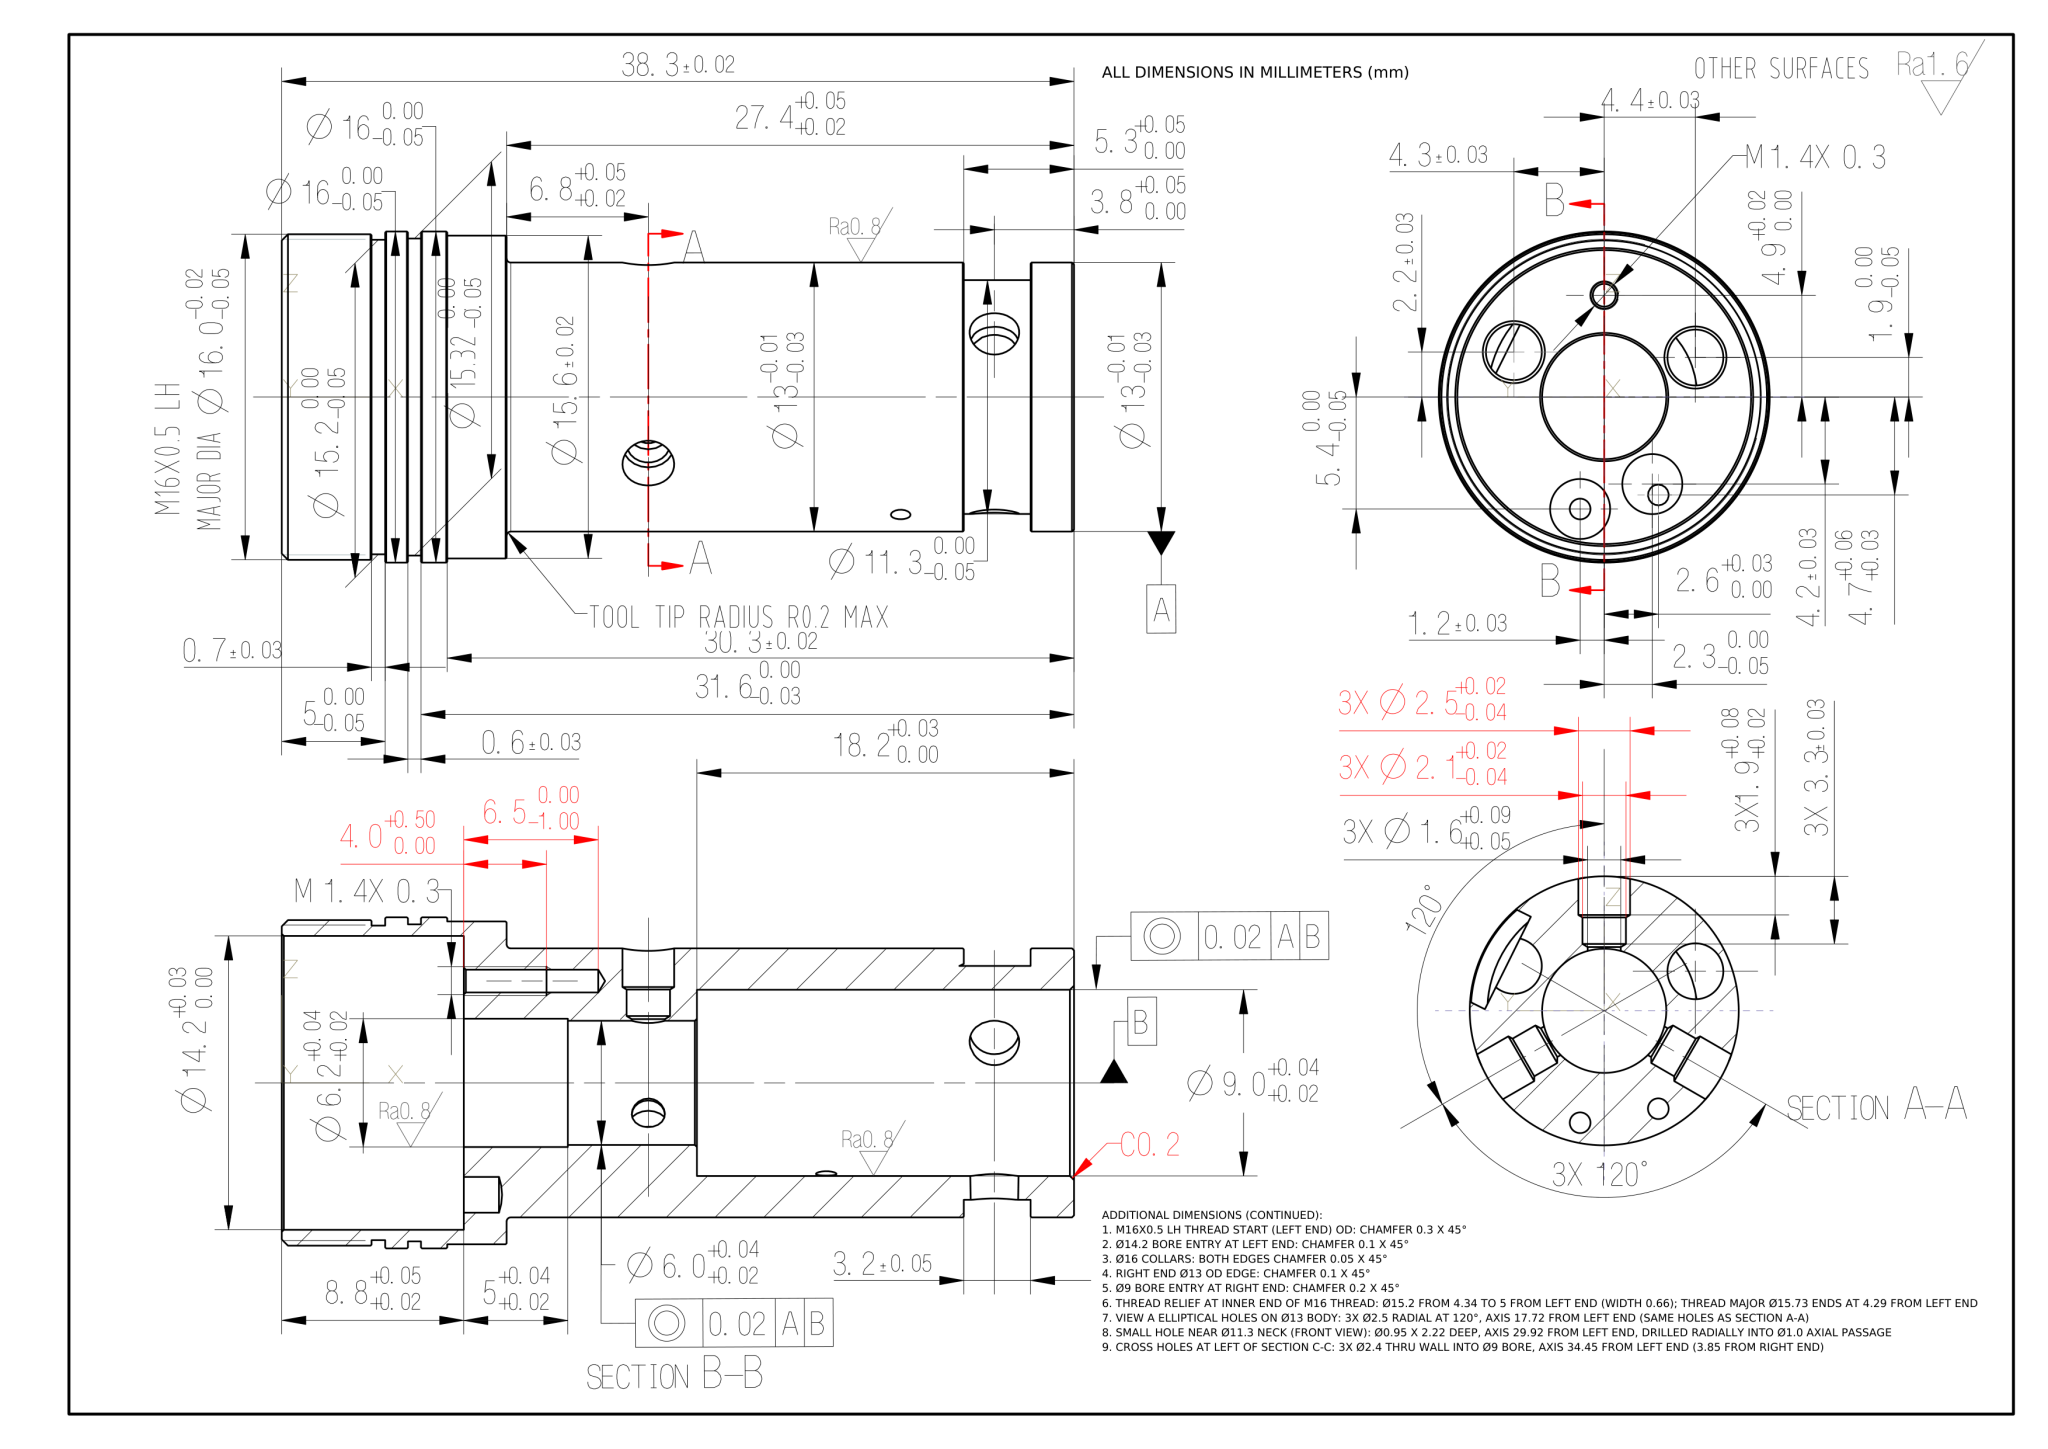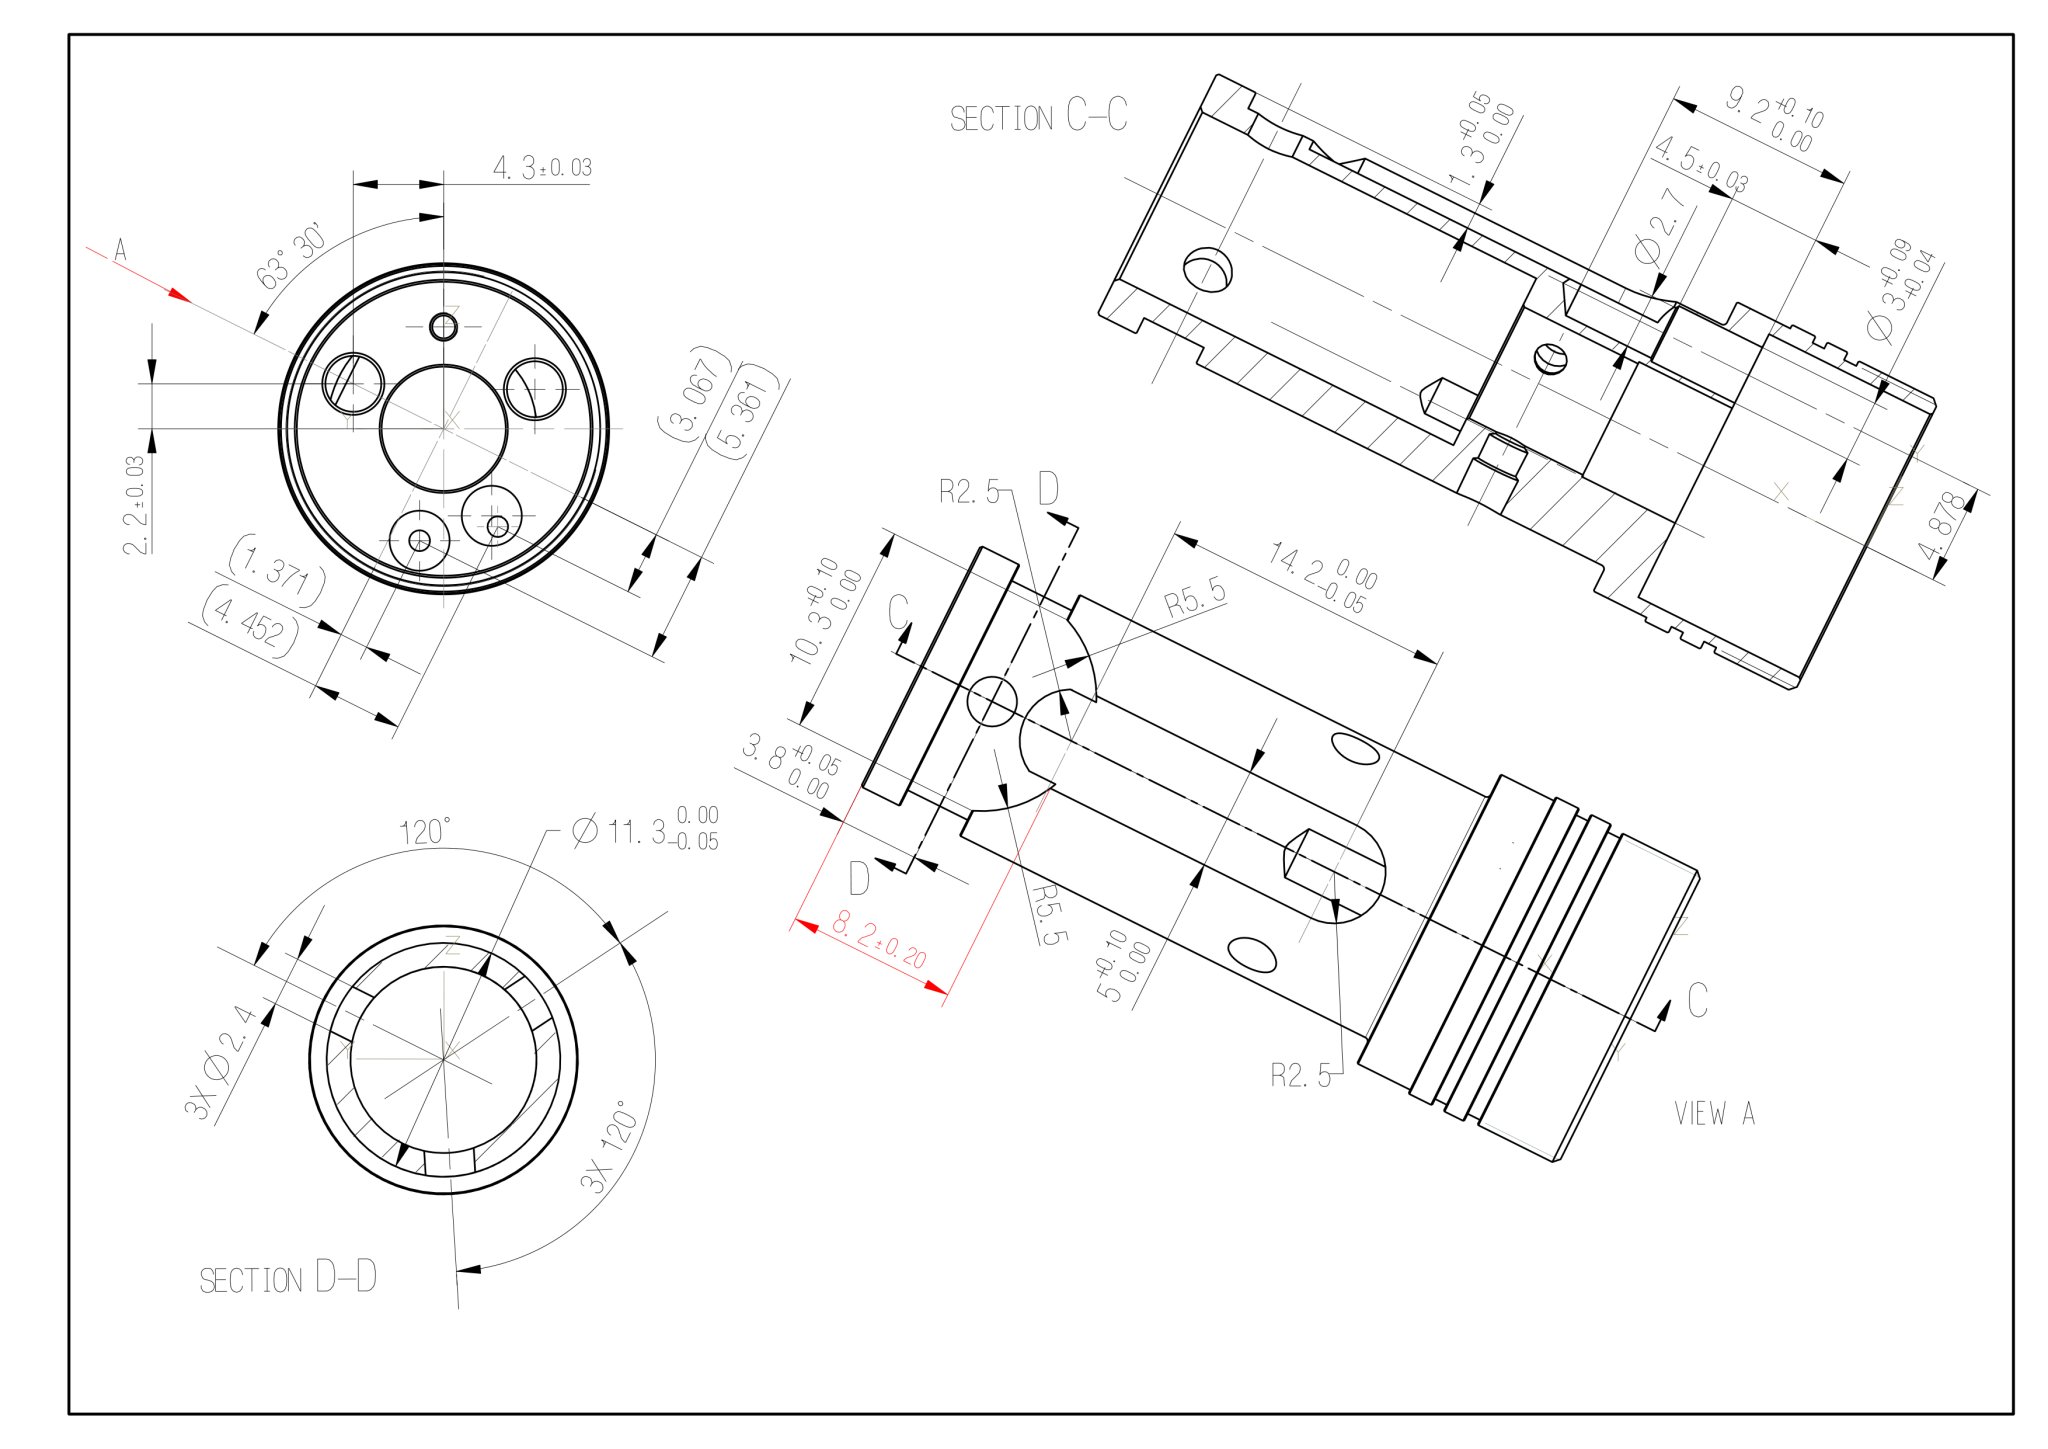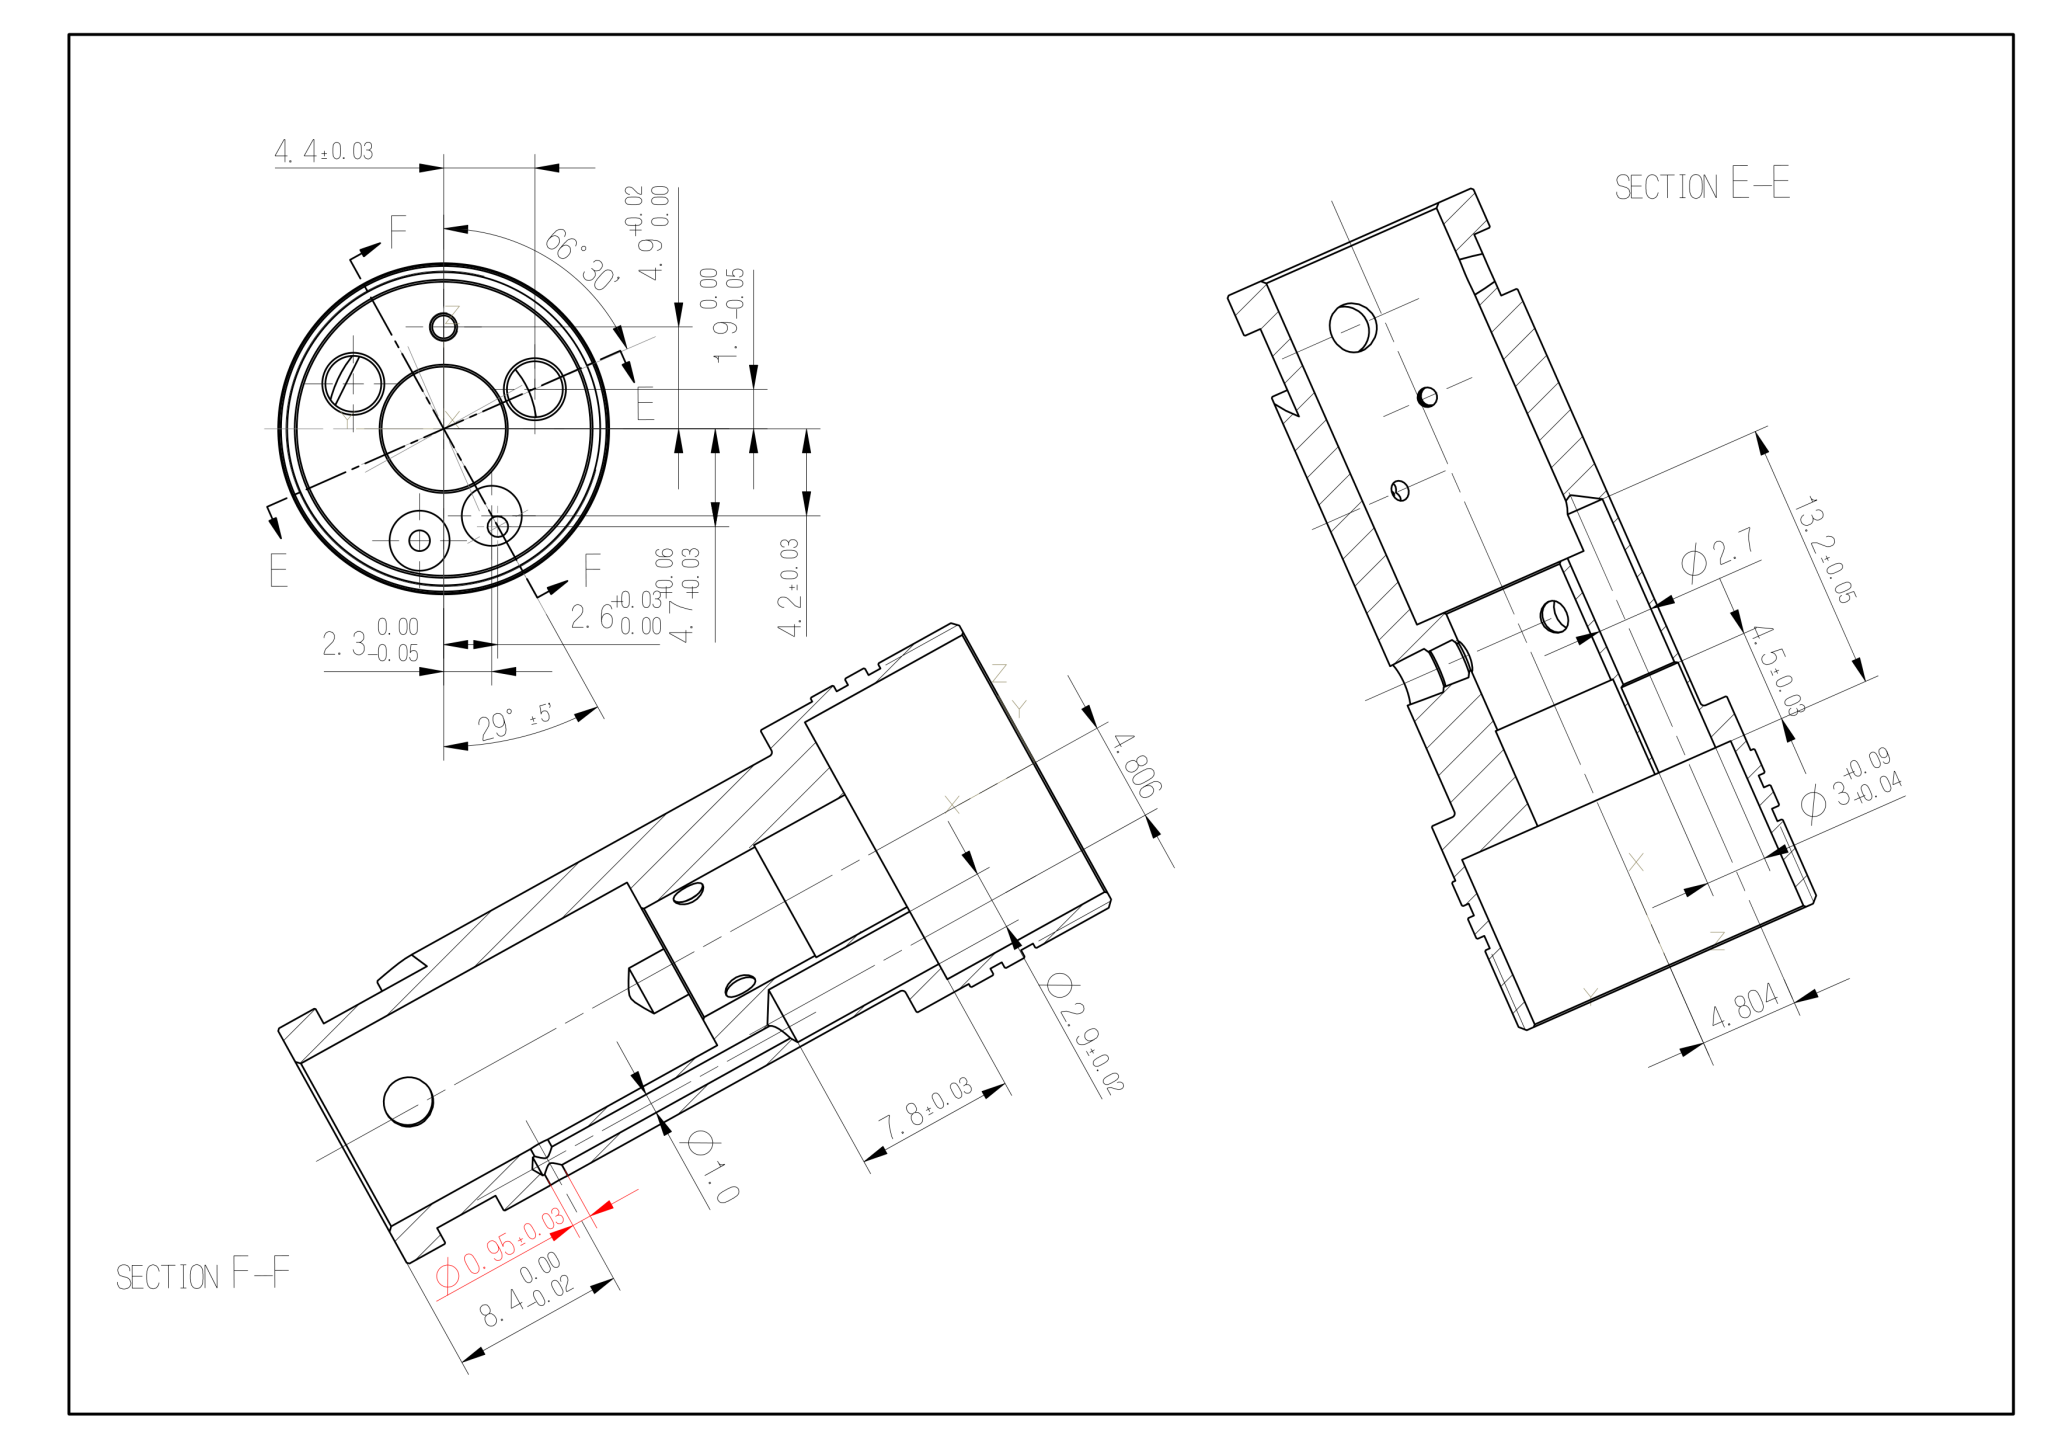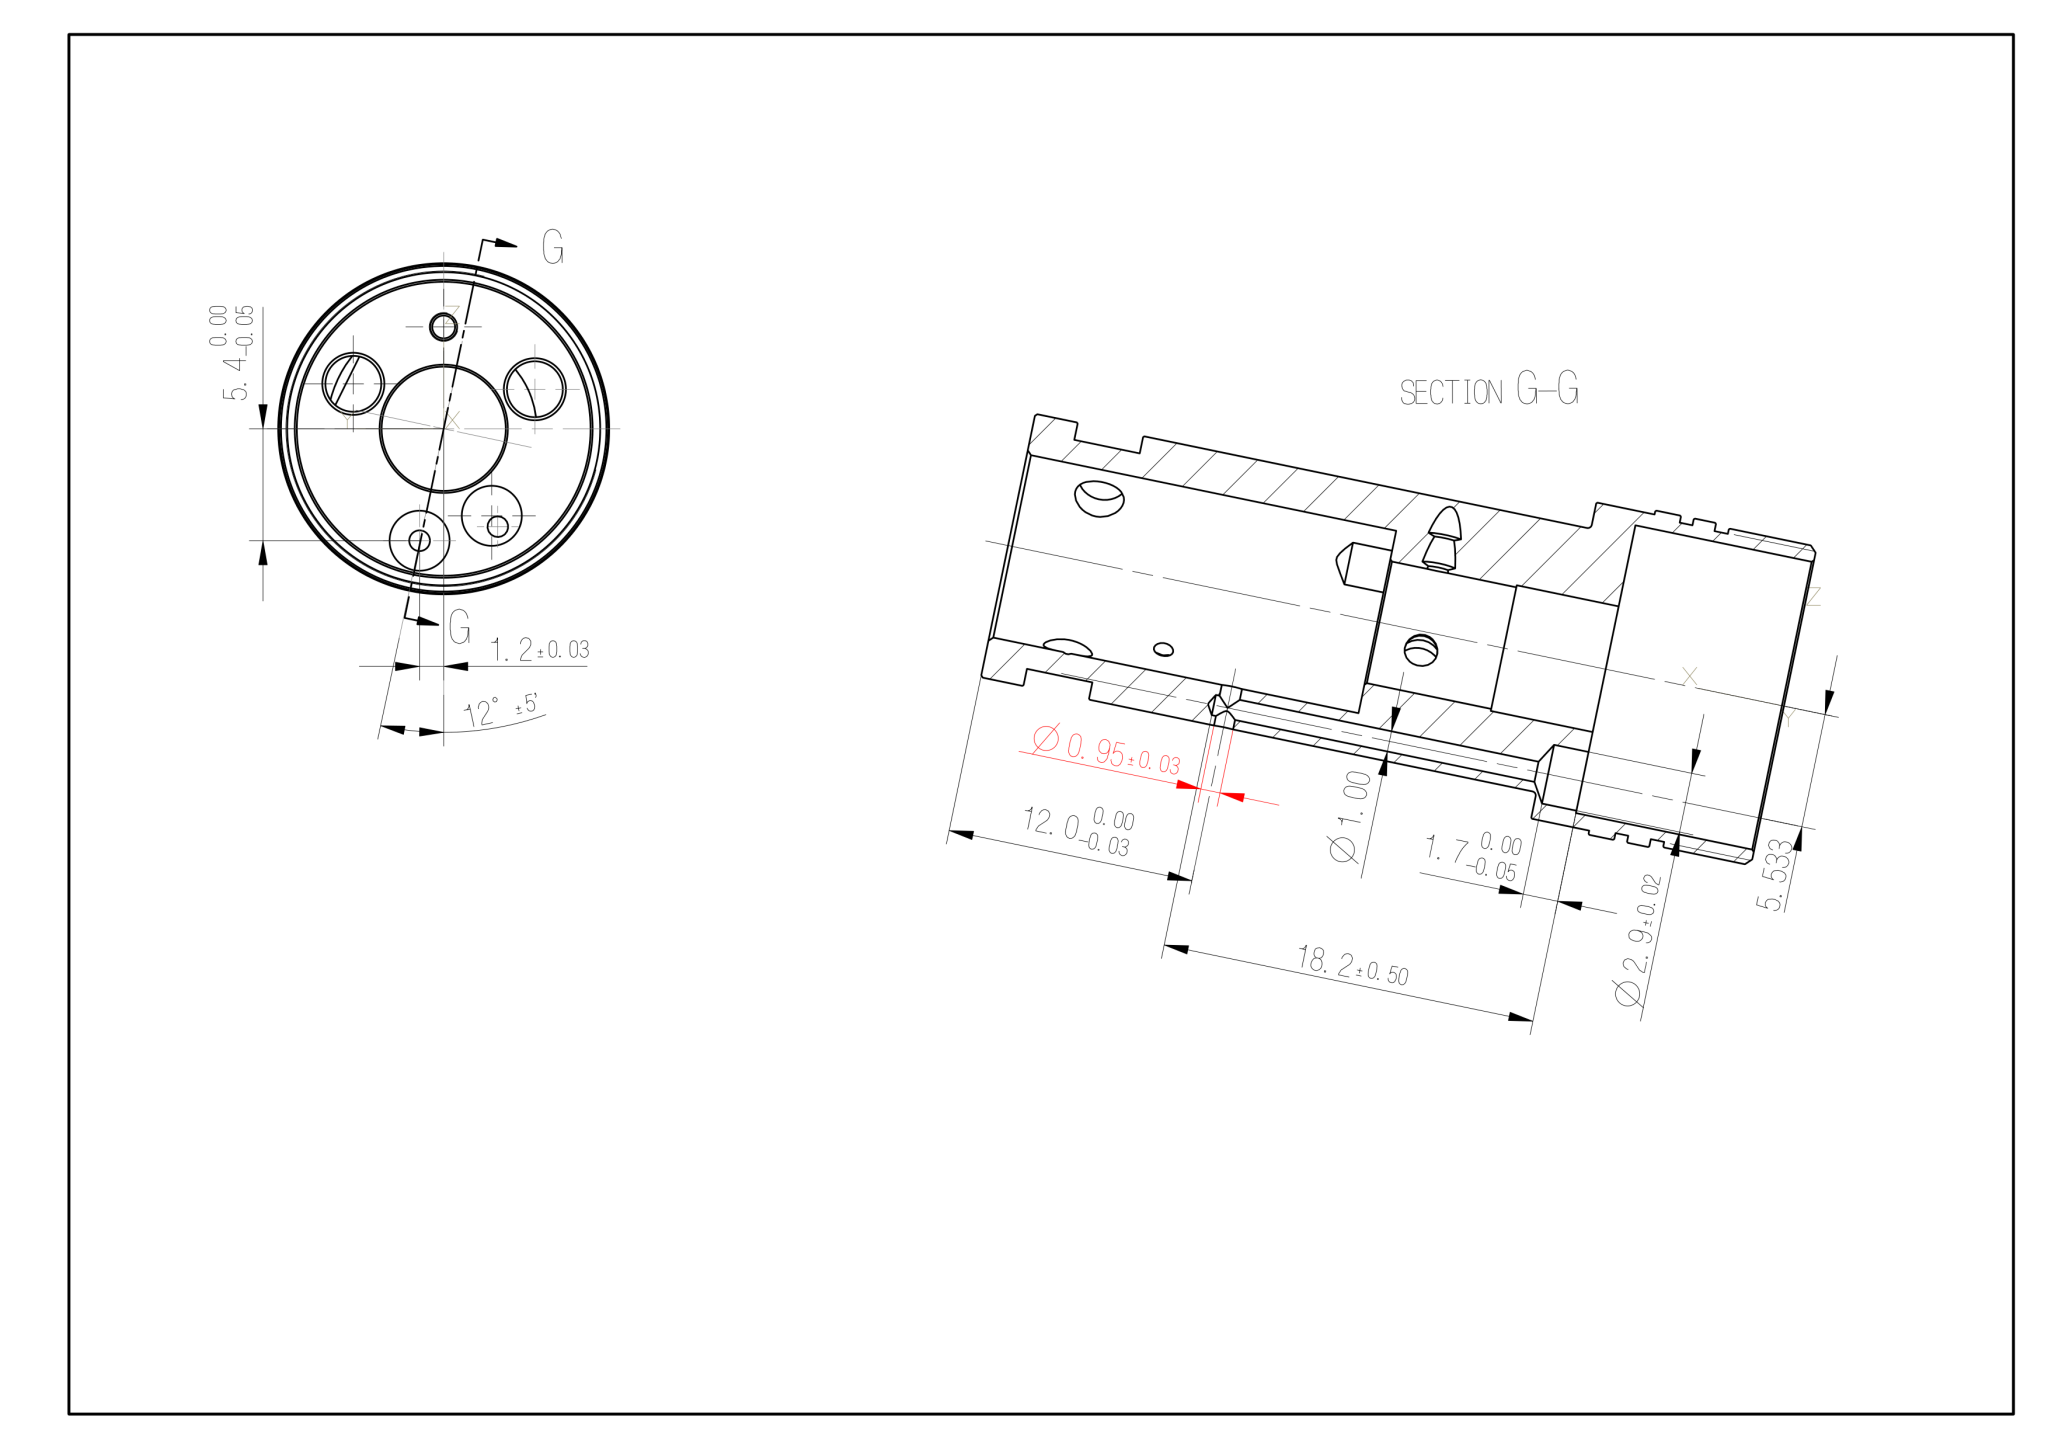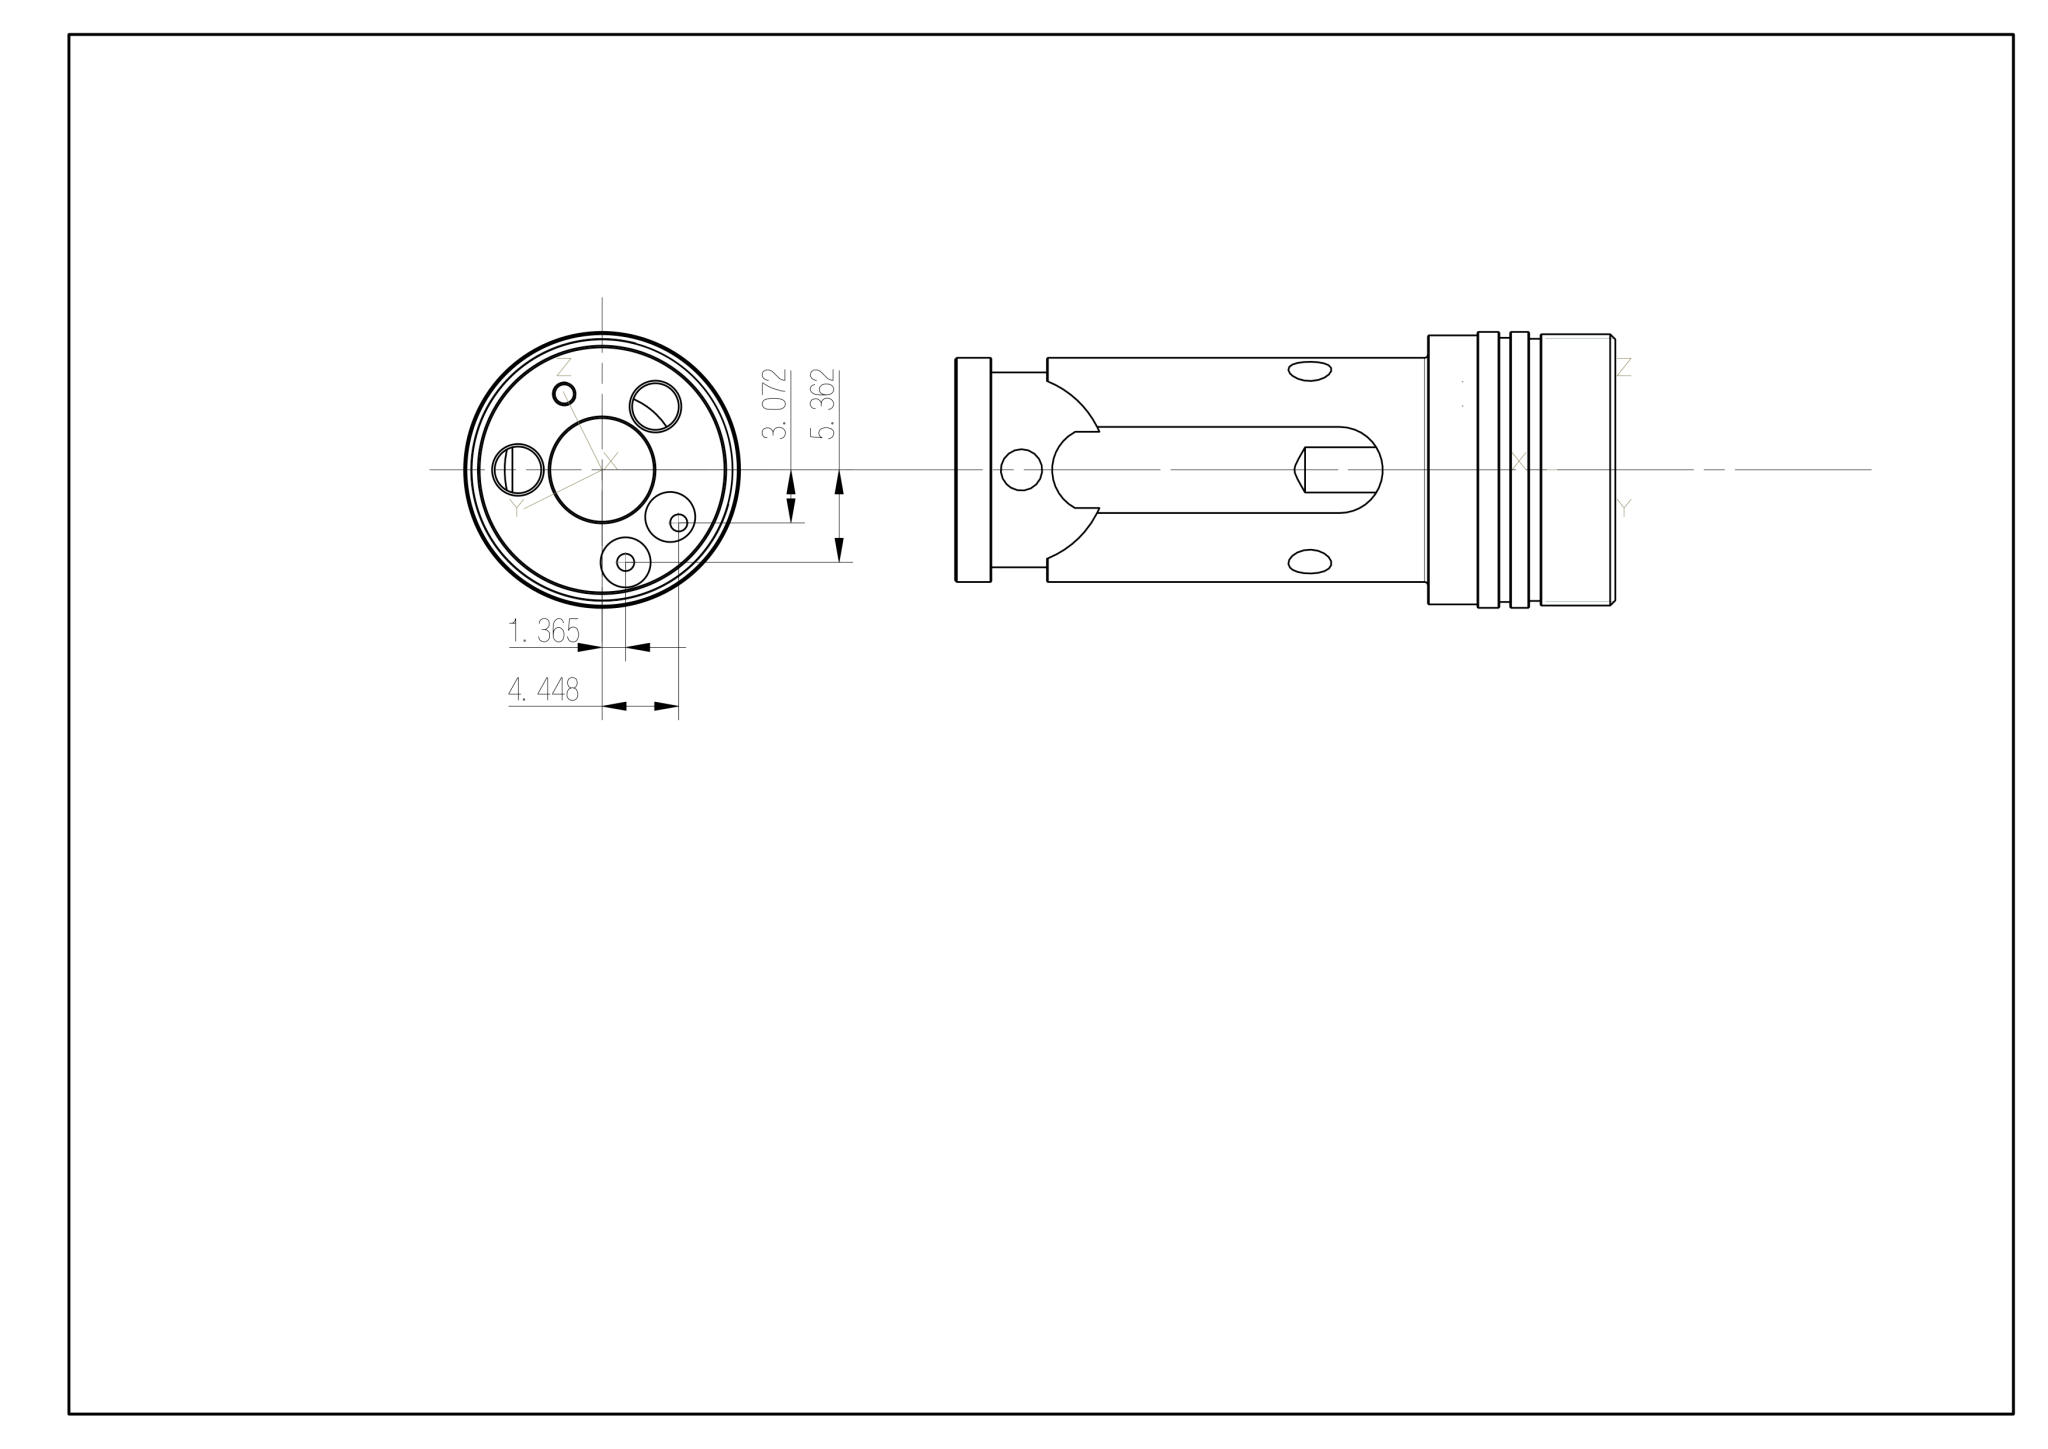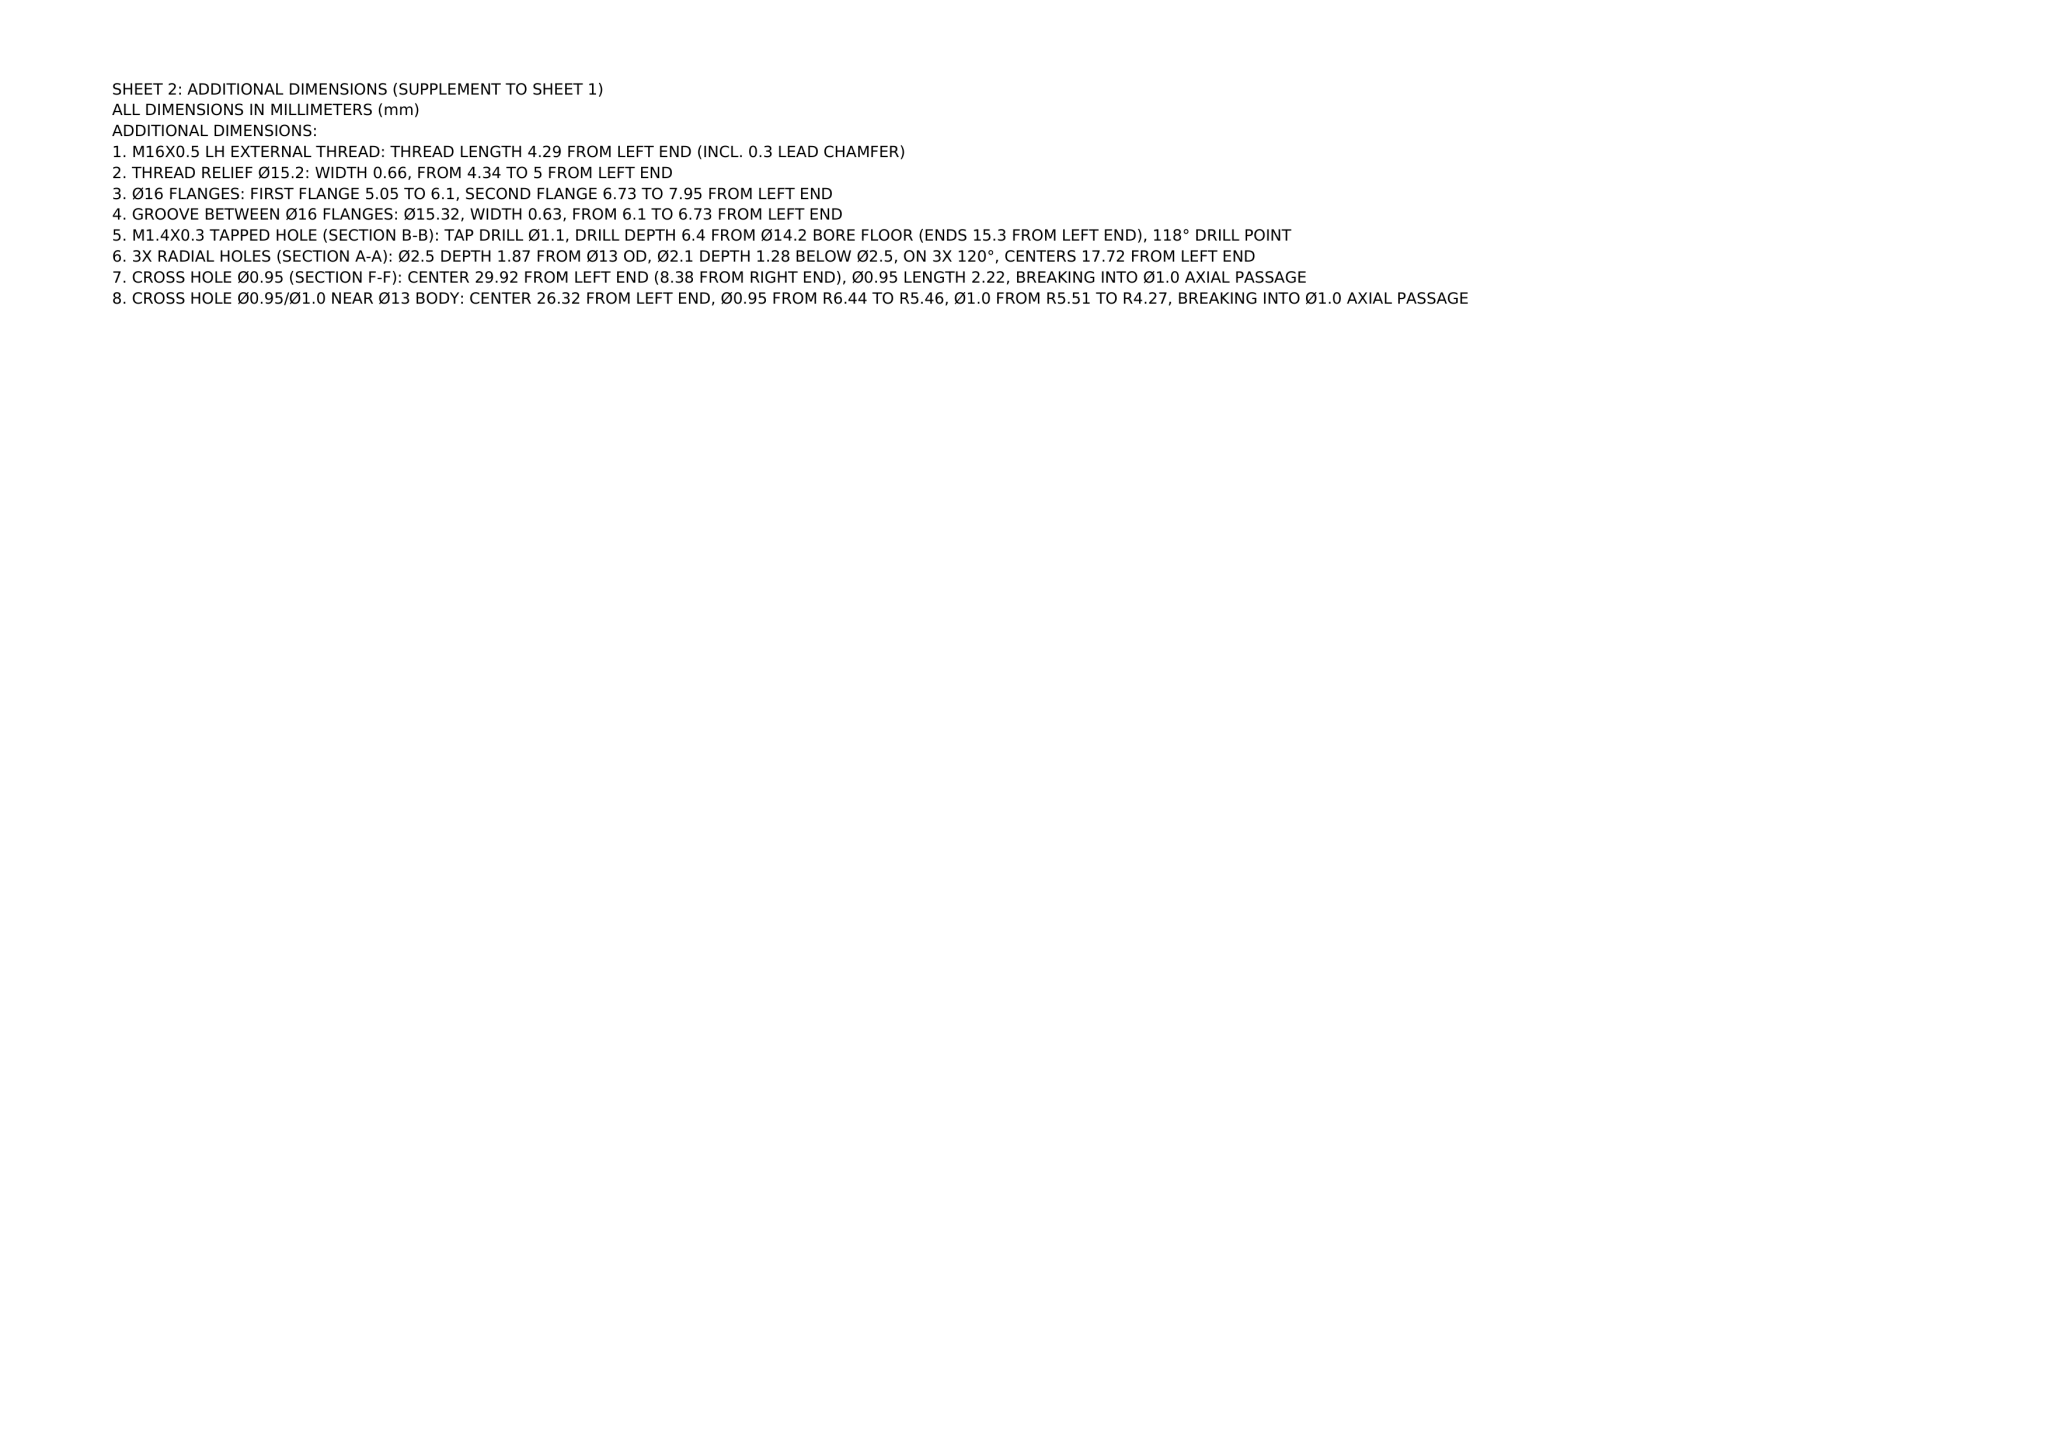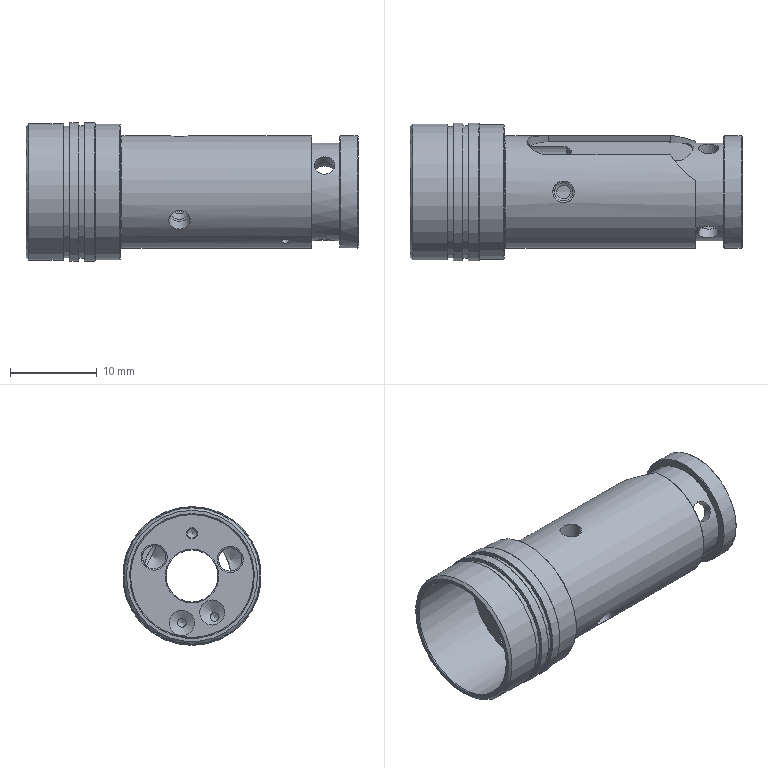Part | NX | mm | 1 solid | 89 faces | box 38.3 x 16 x 16 mm | volume 2351 mm3 | cylinder 43 | cone 29 | plane 16 | torus 1 | commonest cylinder face diameters 1 x4 2.4 x3 0.95 x3 1.6 x3 2.5 x3 2.1 x3 13 x2 16 x2